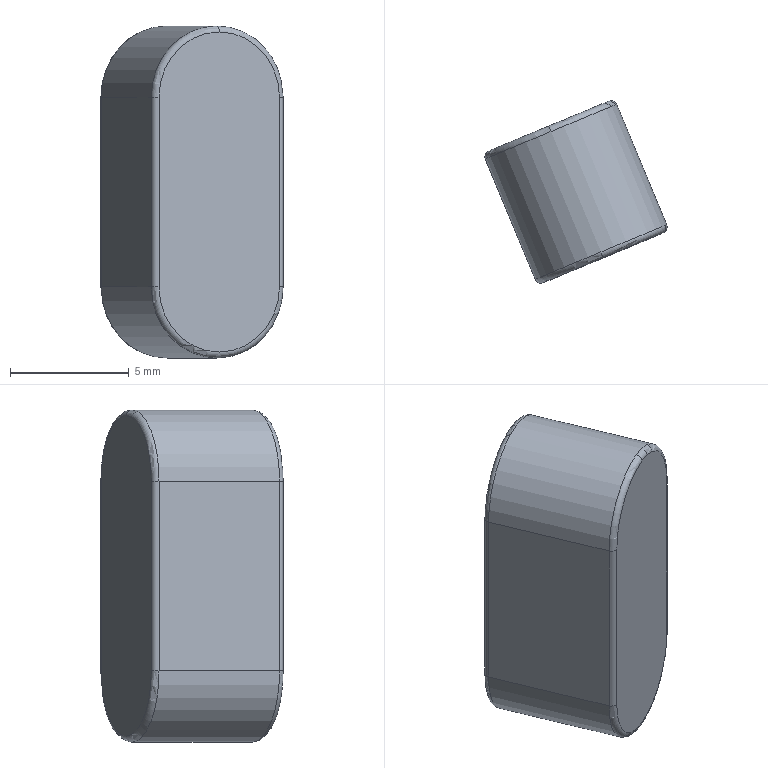Component | NX | GB_T_1096_2003_KEY_A_6X6X14 | 1 solid | 17 faces | box 7.69 x 7.69 x 14 mm | volume 457 mm3 | cylinder 7 | torus 6 | plane 4 | commonest cylinder face diameters 0.5 x4 6 x3
STEP:
#1=CARTESIAN_POINT('',(0.,0.,0.));
#2=DIRECTION('',(0.,0.,1.));
#3=DIRECTION('',(1.,0.,0.));
#4=AXIS2_PLACEMENT_3D('',#1,#2,#3);
#5=CARTESIAN_POINT('',(1.005,16.868,327.723));
#6=VERTEX_POINT('',#5);
#7=CARTESIAN_POINT('',(-1.536,15.814,324.973));
#8=VERTEX_POINT('',#7);
#9=CARTESIAN_POINT('',(1.005,16.868,324.973));
#10=DIRECTION('',(0.383,-0.9237,0.));
#11=DIRECTION('',(0.,0.,1.));
#12=AXIS2_PLACEMENT_3D('',#9,#10,#11);
#13=CIRCLE('',#12,2.75);
#14=CARTESIAN_POINT('',(0.9089,17.099,324.973));
#15=DIRECTION('',(-0.383,0.9237,0.));
#16=DIRECTION('',(0.,0.,-1.));
#17=AXIS2_PLACEMENT_3D('',#14,#15,#16);
#18=TOROIDAL_SURFACE('',#17,2.75,0.25);
#19=CARTESIAN_POINT('',(3.142,4.712));
#20=DIRECTION('',(-1.,-0.));
#21=VECTOR('',#20,1.);
#22=LINE('',#19,#21);
#23=(GEOMETRIC_REPRESENTATION_CONTEXT(2)PARAMETRIC_REPRESENTATION_CONTEXT()REPRESENTATION_CONTEXT('',''));
#24=DEFINITIONAL_REPRESENTATION('',(#22),#23);
#25=PCURVE('',#18,#24);
#26=CARTESIAN_POINT('',(1.005,16.868,316.973));
#27=DIRECTION('',(-0.383,0.9237,0.));
#28=DIRECTION('',(0.,0.,-1.));
#29=AXIS2_PLACEMENT_3D('',#26,#27,#28);
#30=PLANE('',#29);
#31=CARTESIAN_POINT('',(-10.75,0.));
#32=CARTESIAN_POINT('',(-10.75,4.763));
#33=CARTESIAN_POINT('',(-6.625,2.382));
#34=CARTESIAN_POINT('',(-2.5,0.));
#35=CARTESIAN_POINT('',(-6.625,-2.382));
#36=CARTESIAN_POINT('',(-10.75,-4.763));
#37=CARTESIAN_POINT('',(-10.75,0.));
#38=(BOUNDED_CURVE()B_SPLINE_CURVE(2,(#31,#32,#33,#34,#35,#36,#37),.UNSPECIFIED.,.T.,.F.)B_SPLINE_CURVE_WITH_KNOTS((1,2,2,2,2,1),(-2.094,0.,2.094,4.189,6.283,8.378),.UNSPECIFIED.)CURVE()GEOMETRIC_REPRESENTATION_ITEM()RATIONAL_B_SPLINE_CURVE((1.,0.5,1.,0.5,1.,0.5,1.))REPRESENTATION_ITEM(''));
#39=(GEOMETRIC_REPRESENTATION_CONTEXT(2)PARAMETRIC_REPRESENTATION_CONTEXT()REPRESENTATION_CONTEXT('',''));
#40=DEFINITIONAL_REPRESENTATION('',(#38),#39);
#41=PCURVE('',#30,#40);
#42=SURFACE_CURVE('',#13,(#25,#41),.PCURVE_S1.);
#43=EDGE_CURVE('',#6,#8,#42,.T.);
#44=ORIENTED_EDGE('',*,*,#43,.F.);
#45=CARTESIAN_POINT('',(0.9089,17.099,327.973));
#46=VERTEX_POINT('',#45);
#47=CARTESIAN_POINT('',(0.9089,17.099,327.723));
#48=DIRECTION('',(-0.9237,-0.383,0.));
#49=DIRECTION('',(0.383,-0.9237,0.));
#50=AXIS2_PLACEMENT_3D('',#47,#48,#49);
#51=CIRCLE('',#50,0.25);
#52=CARTESIAN_POINT('',(3.142,4.712));
#53=DIRECTION('',(0.,1.));
#54=VECTOR('',#53,1.);
#55=LINE('',#52,#54);
#56=(GEOMETRIC_REPRESENTATION_CONTEXT(2)PARAMETRIC_REPRESENTATION_CONTEXT()REPRESENTATION_CONTEXT('',''));
#57=DEFINITIONAL_REPRESENTATION('',(#55),#56);
#58=PCURVE('',#18,#57);
#59=CARTESIAN_POINT('',(0.9089,17.099,324.973));
#60=DIRECTION('',(-0.383,0.9237,0.));
#61=DIRECTION('',(0.,0.,-1.));
#62=AXIS2_PLACEMENT_3D('',#59,#60,#61);
#63=TOROIDAL_SURFACE('',#62,2.75,0.25);
#64=CARTESIAN_POINT('',(3.142,4.712));
#65=DIRECTION('',(0.,1.));
#66=VECTOR('',#65,1.);
#67=LINE('',#64,#66);
#68=(GEOMETRIC_REPRESENTATION_CONTEXT(2)PARAMETRIC_REPRESENTATION_CONTEXT()REPRESENTATION_CONTEXT('',''));
#69=DEFINITIONAL_REPRESENTATION('',(#67),#68);
#70=PCURVE('',#63,#69);
#71=SURFACE_CURVE('',#51,(#58,#70),.PCURVE_S1.);
#72=EDGE_CURVE('',#6,#46,#71,.T.);
#73=ORIENTED_EDGE('',*,*,#72,.T.);
#74=CARTESIAN_POINT('',(-1.862,15.949,324.973));
#75=VERTEX_POINT('',#74);
#76=CARTESIAN_POINT('',(0.9089,17.099,324.973));
#77=DIRECTION('',(-0.383,0.9237,0.));
#78=DIRECTION('',(0.,0.,1.));
#79=AXIS2_PLACEMENT_3D('',#76,#77,#78);
#80=CIRCLE('',#79,3.);
#81=CARTESIAN_POINT('',(-3.142,6.283));
#82=DIRECTION('',(1.,0.));
#83=VECTOR('',#82,1.);
#84=LINE('',#81,#83);
#85=(GEOMETRIC_REPRESENTATION_CONTEXT(2)PARAMETRIC_REPRESENTATION_CONTEXT()REPRESENTATION_CONTEXT('',''));
#86=DEFINITIONAL_REPRESENTATION('',(#84),#85);
#87=PCURVE('',#18,#86);
#88=CARTESIAN_POINT('',(-1.294,22.41,324.973));
#89=DIRECTION('',(0.383,-0.9237,0.));
#90=DIRECTION('',(0.,0.,1.));
#91=AXIS2_PLACEMENT_3D('',#88,#89,#90);
#92=CYLINDRICAL_SURFACE('',#91,3.);
#93=CARTESIAN_POINT('',(12.566,5.75));
#94=DIRECTION('',(-1.,-0.));
#95=VECTOR('',#94,1.);
#96=LINE('',#93,#95);
#97=(GEOMETRIC_REPRESENTATION_CONTEXT(2)PARAMETRIC_REPRESENTATION_CONTEXT()REPRESENTATION_CONTEXT('',''));
#98=DEFINITIONAL_REPRESENTATION('',(#96),#97);
#99=PCURVE('',#92,#98);
#100=SURFACE_CURVE('',#80,(#87,#99),.PCURVE_S1.);
#101=EDGE_CURVE('',#75,#46,#100,.T.);
#102=ORIENTED_EDGE('',*,*,#101,.F.);
#103=CARTESIAN_POINT('',(-1.631,16.045,324.973));
#104=DIRECTION('',(0.,0.,1.));
#105=DIRECTION('',(0.383,-0.9237,0.));
#106=AXIS2_PLACEMENT_3D('',#103,#104,#105);
#107=CIRCLE('',#106,0.25);
#108=CARTESIAN_POINT('',(1.571,10.996));
#109=DIRECTION('',(0.,-1.));
#110=VECTOR('',#109,1.);
#111=LINE('',#108,#110);
#112=(GEOMETRIC_REPRESENTATION_CONTEXT(2)PARAMETRIC_REPRESENTATION_CONTEXT()REPRESENTATION_CONTEXT('',''));
#113=DEFINITIONAL_REPRESENTATION('',(#111),#112);
#114=PCURVE('',#18,#113);
#115=CARTESIAN_POINT('',(-1.631,16.045,316.973));
#116=DIRECTION('',(0.,0.,1.));
#117=DIRECTION('',(-0.383,0.9237,0.));
#118=AXIS2_PLACEMENT_3D('',#115,#116,#117);
#119=CYLINDRICAL_SURFACE('',#118,0.25);
#120=CARTESIAN_POINT('',(-3.142,8.));
#121=DIRECTION('',(1.,0.));
#122=VECTOR('',#121,1.);
#123=LINE('',#120,#122);
#124=(GEOMETRIC_REPRESENTATION_CONTEXT(2)PARAMETRIC_REPRESENTATION_CONTEXT()REPRESENTATION_CONTEXT('',''));
#125=DEFINITIONAL_REPRESENTATION('',(#123),#124);
#126=PCURVE('',#119,#125);
#127=SURFACE_CURVE('',#107,(#114,#126),.PCURVE_S1.);
#128=EDGE_CURVE('',#75,#8,#127,.T.);
#129=ORIENTED_EDGE('',*,*,#128,.T.);
#130=EDGE_LOOP('',(#44,#73,#102,#129));
#131=FACE_BOUND('',#130,.T.);
#132=ADVANCED_FACE('',(#131),#18,.T.);
#133=CARTESIAN_POINT('',(-1.198,22.179,327.973));
#134=VERTEX_POINT('',#133);
#135=CARTESIAN_POINT('',(-3.969,21.03,324.973));
#136=VERTEX_POINT('',#135);
#137=CARTESIAN_POINT('',(-1.198,22.179,324.973));
#138=DIRECTION('',(0.383,-0.9237,0.));
#139=DIRECTION('',(0.,0.,1.));
#140=AXIS2_PLACEMENT_3D('',#137,#138,#139);
#141=CIRCLE('',#140,3.);
#142=CARTESIAN_POINT('',(-1.198,22.179,324.973));
#143=DIRECTION('',(-0.383,0.9237,0.));
#144=DIRECTION('',(0.,0.,-1.));
#145=AXIS2_PLACEMENT_3D('',#142,#143,#144);
#146=TOROIDAL_SURFACE('',#145,2.75,0.25);
#147=CARTESIAN_POINT('',(3.142,0.));
#148=DIRECTION('',(-1.,0.));
#149=VECTOR('',#148,1.);
#150=LINE('',#147,#149);
#151=(GEOMETRIC_REPRESENTATION_CONTEXT(2)PARAMETRIC_REPRESENTATION_CONTEXT()REPRESENTATION_CONTEXT('',''));
#152=DEFINITIONAL_REPRESENTATION('',(#150),#151);
#153=PCURVE('',#146,#152);
#154=CARTESIAN_POINT('',(6.283,0.25));
#155=DIRECTION('',(1.,-0.));
#156=VECTOR('',#155,1.);
#157=LINE('',#154,#156);
#158=(GEOMETRIC_REPRESENTATION_CONTEXT(2)PARAMETRIC_REPRESENTATION_CONTEXT()REPRESENTATION_CONTEXT('',''));
#159=DEFINITIONAL_REPRESENTATION('',(#157),#158);
#160=PCURVE('',#92,#159);
#161=SURFACE_CURVE('',#141,(#153,#160),.PCURVE_S1.);
#162=EDGE_CURVE('',#134,#136,#161,.T.);
#163=ORIENTED_EDGE('',*,*,#162,.F.);
#164=CARTESIAN_POINT('',(-1.294,22.41,327.723));
#165=VERTEX_POINT('',#164);
#166=CARTESIAN_POINT('',(-1.198,22.179,327.723));
#167=DIRECTION('',(-0.9237,-0.383,0.));
#168=DIRECTION('',(0.383,-0.9237,0.));
#169=AXIS2_PLACEMENT_3D('',#166,#167,#168);
#170=CIRCLE('',#169,0.25);
#171=CARTESIAN_POINT('',(3.142,-1.571));
#172=DIRECTION('',(0.,1.));
#173=VECTOR('',#172,1.);
#174=LINE('',#171,#173);
#175=(GEOMETRIC_REPRESENTATION_CONTEXT(2)PARAMETRIC_REPRESENTATION_CONTEXT()REPRESENTATION_CONTEXT('',''));
#176=DEFINITIONAL_REPRESENTATION('',(#174),#175);
#177=PCURVE('',#146,#176);
#178=CARTESIAN_POINT('',(-1.198,22.179,324.973));
#179=DIRECTION('',(-0.383,0.9237,0.));
#180=DIRECTION('',(0.,0.,-1.));
#181=AXIS2_PLACEMENT_3D('',#178,#179,#180);
#182=TOROIDAL_SURFACE('',#181,2.75,0.25);
#183=CARTESIAN_POINT('',(3.142,-1.571));
#184=DIRECTION('',(0.,1.));
#185=VECTOR('',#184,1.);
#186=LINE('',#183,#185);
#187=(GEOMETRIC_REPRESENTATION_CONTEXT(2)PARAMETRIC_REPRESENTATION_CONTEXT()REPRESENTATION_CONTEXT('',''));
#188=DEFINITIONAL_REPRESENTATION('',(#186),#187);
#189=PCURVE('',#182,#188);
#190=SURFACE_CURVE('',#170,(#177,#189),.PCURVE_S1.);
#191=EDGE_CURVE('',#134,#165,#190,.T.);
#192=ORIENTED_EDGE('',*,*,#191,.T.);
#193=CARTESIAN_POINT('',(-3.834,21.357,324.973));
#194=VERTEX_POINT('',#193);
#195=CARTESIAN_POINT('',(-1.294,22.41,324.973));
#196=DIRECTION('',(-0.383,0.9237,0.));
#197=DIRECTION('',(0.,0.,1.));
#198=AXIS2_PLACEMENT_3D('',#195,#196,#197);
#199=CIRCLE('',#198,2.75);
#200=CARTESIAN_POINT('',(-3.142,1.571));
#201=DIRECTION('',(1.,-0.));
#202=VECTOR('',#201,1.);
#203=LINE('',#200,#202);
#204=(GEOMETRIC_REPRESENTATION_CONTEXT(2)PARAMETRIC_REPRESENTATION_CONTEXT()REPRESENTATION_CONTEXT('',''));
#205=DEFINITIONAL_REPRESENTATION('',(#203),#204);
#206=PCURVE('',#146,#205);
#207=CARTESIAN_POINT('',(-1.294,22.41,316.973));
#208=DIRECTION('',(-0.383,0.9237,0.));
#209=DIRECTION('',(0.,0.,-1.));
#210=AXIS2_PLACEMENT_3D('',#207,#208,#209);
#211=PLANE('',#210);
#212=CARTESIAN_POINT('',(-8.,0.));
#213=DIRECTION('',(-1.,0.));
#214=AXIS2_PLACEMENT_2D('',#212,#213);
#215=CIRCLE('',#214,2.75);
#216=(GEOMETRIC_REPRESENTATION_CONTEXT(2)PARAMETRIC_REPRESENTATION_CONTEXT()REPRESENTATION_CONTEXT('',''));
#217=DEFINITIONAL_REPRESENTATION('',(#215),#216);
#218=PCURVE('',#211,#217);
#219=SURFACE_CURVE('',#199,(#206,#218),.PCURVE_S1.);
#220=EDGE_CURVE('',#194,#165,#219,.T.);
#221=ORIENTED_EDGE('',*,*,#220,.F.);
#222=CARTESIAN_POINT('',(-3.738,21.126,324.973));
#223=DIRECTION('',(0.,0.,1.));
#224=DIRECTION('',(0.383,-0.9237,0.));
#225=AXIS2_PLACEMENT_3D('',#222,#223,#224);
#226=CIRCLE('',#225,0.25);
#227=CARTESIAN_POINT('',(1.571,4.712));
#228=DIRECTION('',(0.,-1.));
#229=VECTOR('',#228,1.);
#230=LINE('',#227,#229);
#231=(GEOMETRIC_REPRESENTATION_CONTEXT(2)PARAMETRIC_REPRESENTATION_CONTEXT()REPRESENTATION_CONTEXT('',''));
#232=DEFINITIONAL_REPRESENTATION('',(#230),#231);
#233=PCURVE('',#146,#232);
#234=CARTESIAN_POINT('',(-3.738,21.126,316.973));
#235=DIRECTION('',(0.,0.,-1.));
#236=DIRECTION('',(0.383,-0.9237,0.));
#237=AXIS2_PLACEMENT_3D('',#234,#235,#236);
#238=CYLINDRICAL_SURFACE('',#237,0.25);
#239=CARTESIAN_POINT('',(6.283,-8.));
#240=DIRECTION('',(-1.,0.));
#241=VECTOR('',#240,1.);
#242=LINE('',#239,#241);
#243=(GEOMETRIC_REPRESENTATION_CONTEXT(2)PARAMETRIC_REPRESENTATION_CONTEXT()REPRESENTATION_CONTEXT('',''));
#244=DEFINITIONAL_REPRESENTATION('',(#242),#243);
#245=PCURVE('',#238,#244);
#246=SURFACE_CURVE('',#226,(#233,#245),.PCURVE_S1.);
#247=EDGE_CURVE('',#194,#136,#246,.T.);
#248=ORIENTED_EDGE('',*,*,#247,.T.);
#249=EDGE_LOOP('',(#163,#192,#221,#248));
#250=FACE_BOUND('',#249,.T.);
#251=ADVANCED_FACE('',(#250),#146,.T.);
#252=CARTESIAN_POINT('',(-3.969,21.03,316.973));
#253=VERTEX_POINT('',#252);
#254=CARTESIAN_POINT('',(-1.198,22.179,313.973));
#255=VERTEX_POINT('',#254);
#256=CARTESIAN_POINT('',(-1.198,22.179,316.973));
#257=DIRECTION('',(0.383,-0.9237,0.));
#258=DIRECTION('',(0.,0.,1.));
#259=AXIS2_PLACEMENT_3D('',#256,#257,#258);
#260=CIRCLE('',#259,3.);
#261=CARTESIAN_POINT('',(-1.294,22.41,316.973));
#262=DIRECTION('',(0.383,-0.9237,0.));
#263=DIRECTION('',(0.,0.,1.));
#264=AXIS2_PLACEMENT_3D('',#261,#262,#263);
#265=CYLINDRICAL_SURFACE('',#264,3.);
#266=CARTESIAN_POINT('',(-0.,0.25));
#267=DIRECTION('',(1.,0.));
#268=VECTOR('',#267,1.);
#269=LINE('',#266,#268);
#270=(GEOMETRIC_REPRESENTATION_CONTEXT(2)PARAMETRIC_REPRESENTATION_CONTEXT()REPRESENTATION_CONTEXT('',''));
#271=DEFINITIONAL_REPRESENTATION('',(#269),#270);
#272=PCURVE('',#265,#271);
#273=CARTESIAN_POINT('',(-1.198,22.179,316.973));
#274=DIRECTION('',(-0.383,0.9237,0.));
#275=DIRECTION('',(0.,0.,-1.));
#276=AXIS2_PLACEMENT_3D('',#273,#274,#275);
#277=TOROIDAL_SURFACE('',#276,2.75,0.25);
#278=CARTESIAN_POINT('',(9.425,0.));
#279=DIRECTION('',(-1.,0.));
#280=VECTOR('',#279,1.);
#281=LINE('',#278,#280);
#282=(GEOMETRIC_REPRESENTATION_CONTEXT(2)PARAMETRIC_REPRESENTATION_CONTEXT()REPRESENTATION_CONTEXT('',''));
#283=DEFINITIONAL_REPRESENTATION('',(#281),#282);
#284=PCURVE('',#277,#283);
#285=SURFACE_CURVE('',#260,(#272,#284),.PCURVE_S1.);
#286=EDGE_CURVE('',#253,#255,#285,.T.);
#287=ORIENTED_EDGE('',*,*,#286,.T.);
#288=CARTESIAN_POINT('',(0.9089,17.099,313.973));
#289=VERTEX_POINT('',#288);
#290=CARTESIAN_POINT('',(-1.294,22.41,313.973));
#291=DIRECTION('',(0.383,-0.9237,0.));
#292=VECTOR('',#291,1.);
#293=LINE('',#290,#292);
#294=CARTESIAN_POINT('',(3.142,0.));
#295=DIRECTION('',(0.,1.));
#296=VECTOR('',#295,1.);
#297=LINE('',#294,#296);
#298=(GEOMETRIC_REPRESENTATION_CONTEXT(2)PARAMETRIC_REPRESENTATION_CONTEXT()REPRESENTATION_CONTEXT('',''));
#299=DEFINITIONAL_REPRESENTATION('',(#297),#298);
#300=PCURVE('',#265,#299);
#301=CARTESIAN_POINT('',(-1.294,22.41,316.973));
#302=DIRECTION('',(0.383,-0.9237,0.));
#303=DIRECTION('',(0.,0.,1.));
#304=AXIS2_PLACEMENT_3D('',#301,#302,#303);
#305=CYLINDRICAL_SURFACE('',#304,3.);
#306=CARTESIAN_POINT('',(3.142,0.));
#307=DIRECTION('',(0.,1.));
#308=VECTOR('',#307,1.);
#309=LINE('',#306,#308);
#310=(GEOMETRIC_REPRESENTATION_CONTEXT(2)PARAMETRIC_REPRESENTATION_CONTEXT()REPRESENTATION_CONTEXT('',''));
#311=DEFINITIONAL_REPRESENTATION('',(#309),#310);
#312=PCURVE('',#305,#311);
#313=SURFACE_CURVE('',#293,(#300,#312),.PCURVE_S1.);
#314=EDGE_CURVE('',#255,#289,#313,.T.);
#315=ORIENTED_EDGE('',*,*,#314,.T.);
#316=CARTESIAN_POINT('',(-1.862,15.949,316.973));
#317=VERTEX_POINT('',#316);
#318=CARTESIAN_POINT('',(0.9089,17.099,316.973));
#319=DIRECTION('',(-0.383,0.9237,0.));
#320=DIRECTION('',(0.,0.,1.));
#321=AXIS2_PLACEMENT_3D('',#318,#319,#320);
#322=CIRCLE('',#321,3.);
#323=CARTESIAN_POINT('',(6.283,5.75));
#324=DIRECTION('',(-1.,0.));
#325=VECTOR('',#324,1.);
#326=LINE('',#323,#325);
#327=(GEOMETRIC_REPRESENTATION_CONTEXT(2)PARAMETRIC_REPRESENTATION_CONTEXT()REPRESENTATION_CONTEXT('',''));
#328=DEFINITIONAL_REPRESENTATION('',(#326),#327);
#329=PCURVE('',#265,#328);
#330=CARTESIAN_POINT('',(0.9089,17.099,316.973));
#331=DIRECTION('',(-0.383,0.9237,0.));
#332=DIRECTION('',(0.,0.,-1.));
#333=AXIS2_PLACEMENT_3D('',#330,#331,#332);
#334=TOROIDAL_SURFACE('',#333,2.75,0.25);
#335=CARTESIAN_POINT('',(3.142,6.283));
#336=DIRECTION('',(1.,0.));
#337=VECTOR('',#336,1.);
#338=LINE('',#335,#337);
#339=(GEOMETRIC_REPRESENTATION_CONTEXT(2)PARAMETRIC_REPRESENTATION_CONTEXT()REPRESENTATION_CONTEXT('',''));
#340=DEFINITIONAL_REPRESENTATION('',(#338),#339);
#341=PCURVE('',#334,#340);
#342=SURFACE_CURVE('',#322,(#329,#341),.PCURVE_S1.);
#343=EDGE_CURVE('',#289,#317,#342,.T.);
#344=ORIENTED_EDGE('',*,*,#343,.T.);
#345=CARTESIAN_POINT('',(-4.065,21.261,316.973));
#346=DIRECTION('',(0.383,-0.9237,0.));
#347=VECTOR('',#346,1.);
#348=LINE('',#345,#347);
#349=CARTESIAN_POINT('',(1.571,-0.));
#350=DIRECTION('',(0.,1.));
#351=VECTOR('',#350,1.);
#352=LINE('',#349,#351);
#353=(GEOMETRIC_REPRESENTATION_CONTEXT(2)PARAMETRIC_REPRESENTATION_CONTEXT()REPRESENTATION_CONTEXT('',''));
#354=DEFINITIONAL_REPRESENTATION('',(#352),#353);
#355=PCURVE('',#265,#354);
#356=CARTESIAN_POINT('',(-4.065,21.261,316.973));
#357=DIRECTION('',(0.9237,0.383,0.));
#358=DIRECTION('',(0.383,-0.9237,0.));
#359=AXIS2_PLACEMENT_3D('',#356,#357,#358);
#360=PLANE('',#359);
#361=CARTESIAN_POINT('',(0.,0.));
#362=DIRECTION('',(1.,0.));
#363=VECTOR('',#362,1.);
#364=LINE('',#361,#363);
#365=(GEOMETRIC_REPRESENTATION_CONTEXT(2)PARAMETRIC_REPRESENTATION_CONTEXT()REPRESENTATION_CONTEXT('',''));
#366=DEFINITIONAL_REPRESENTATION('',(#364),#365);
#367=PCURVE('',#360,#366);
#368=SURFACE_CURVE('',#348,(#355,#367),.PCURVE_S1.);
#369=EDGE_CURVE('',#253,#317,#368,.T.);
#370=ORIENTED_EDGE('',*,*,#369,.F.);
#371=EDGE_LOOP('',(#287,#315,#344,#370));
#372=FACE_BOUND('',#371,.T.);
#373=ADVANCED_FACE('',(#372),#265,.T.);
#374=ORIENTED_EDGE('',*,*,#314,.F.);
#375=CARTESIAN_POINT('',(1.573,23.328,316.973));
#376=VERTEX_POINT('',#375);
#377=CARTESIAN_POINT('',(-1.198,22.179,316.973));
#378=DIRECTION('',(0.383,-0.9237,0.));
#379=DIRECTION('',(0.,0.,1.));
#380=AXIS2_PLACEMENT_3D('',#377,#378,#379);
#381=CIRCLE('',#380,3.);
#382=CARTESIAN_POINT('',(-0.,0.25));
#383=DIRECTION('',(1.,0.));
#384=VECTOR('',#383,1.);
#385=LINE('',#382,#384);
#386=(GEOMETRIC_REPRESENTATION_CONTEXT(2)PARAMETRIC_REPRESENTATION_CONTEXT()REPRESENTATION_CONTEXT('',''));
#387=DEFINITIONAL_REPRESENTATION('',(#385),#386);
#388=PCURVE('',#305,#387);
#389=CARTESIAN_POINT('',(9.425,0.));
#390=DIRECTION('',(-1.,0.));
#391=VECTOR('',#390,1.);
#392=LINE('',#389,#391);
#393=(GEOMETRIC_REPRESENTATION_CONTEXT(2)PARAMETRIC_REPRESENTATION_CONTEXT()REPRESENTATION_CONTEXT('',''));
#394=DEFINITIONAL_REPRESENTATION('',(#392),#393);
#395=PCURVE('',#277,#394);
#396=SURFACE_CURVE('',#381,(#388,#395),.PCURVE_S1.);
#397=EDGE_CURVE('',#255,#376,#396,.T.);
#398=ORIENTED_EDGE('',*,*,#397,.T.);
#399=CARTESIAN_POINT('',(3.68,18.248,316.973));
#400=VERTEX_POINT('',#399);
#401=CARTESIAN_POINT('',(1.478,23.559,316.973));
#402=DIRECTION('',(0.383,-0.9237,0.));
#403=VECTOR('',#402,1.);
#404=LINE('',#401,#403);
#405=CARTESIAN_POINT('',(4.712,0.));
#406=DIRECTION('',(0.,1.));
#407=VECTOR('',#406,1.);
#408=LINE('',#405,#407);
#409=(GEOMETRIC_REPRESENTATION_CONTEXT(2)PARAMETRIC_REPRESENTATION_CONTEXT()REPRESENTATION_CONTEXT('',''));
#410=DEFINITIONAL_REPRESENTATION('',(#408),#409);
#411=PCURVE('',#305,#410);
#412=CARTESIAN_POINT('',(1.478,23.559,316.973));
#413=DIRECTION('',(-0.9237,-0.383,0.));
#414=DIRECTION('',(-0.383,0.9237,0.));
#415=AXIS2_PLACEMENT_3D('',#412,#413,#414);
#416=PLANE('',#415);
#417=CARTESIAN_POINT('',(0.,0.));
#418=DIRECTION('',(-1.,0.));
#419=VECTOR('',#418,1.);
#420=LINE('',#417,#419);
#421=(GEOMETRIC_REPRESENTATION_CONTEXT(2)PARAMETRIC_REPRESENTATION_CONTEXT()REPRESENTATION_CONTEXT('',''));
#422=DEFINITIONAL_REPRESENTATION('',(#420),#421);
#423=PCURVE('',#416,#422);
#424=SURFACE_CURVE('',#404,(#411,#423),.PCURVE_S1.);
#425=EDGE_CURVE('',#376,#400,#424,.T.);
#426=ORIENTED_EDGE('',*,*,#425,.T.);
#427=CARTESIAN_POINT('',(0.9089,17.099,316.973));
#428=DIRECTION('',(-0.383,0.9237,0.));
#429=DIRECTION('',(0.,0.,1.));
#430=AXIS2_PLACEMENT_3D('',#427,#428,#429);
#431=CIRCLE('',#430,3.);
#432=CARTESIAN_POINT('',(6.283,5.75));
#433=DIRECTION('',(-1.,0.));
#434=VECTOR('',#433,1.);
#435=LINE('',#432,#434);
#436=(GEOMETRIC_REPRESENTATION_CONTEXT(2)PARAMETRIC_REPRESENTATION_CONTEXT()REPRESENTATION_CONTEXT('',''));
#437=DEFINITIONAL_REPRESENTATION('',(#435),#436);
#438=PCURVE('',#305,#437);
#439=CARTESIAN_POINT('',(3.142,6.283));
#440=DIRECTION('',(1.,0.));
#441=VECTOR('',#440,1.);
#442=LINE('',#439,#441);
#443=(GEOMETRIC_REPRESENTATION_CONTEXT(2)PARAMETRIC_REPRESENTATION_CONTEXT()REPRESENTATION_CONTEXT('',''));
#444=DEFINITIONAL_REPRESENTATION('',(#442),#443);
#445=PCURVE('',#334,#444);
#446=SURFACE_CURVE('',#431,(#438,#445),.PCURVE_S1.);
#447=EDGE_CURVE('',#400,#289,#446,.T.);
#448=ORIENTED_EDGE('',*,*,#447,.T.);
#449=EDGE_LOOP('',(#374,#398,#426,#448));
#450=FACE_BOUND('',#449,.T.);
#451=ADVANCED_FACE('',(#450),#305,.T.);
#452=CARTESIAN_POINT('',(-4.065,21.261,324.973));
#453=DIRECTION('',(0.383,-0.9237,0.));
#454=VECTOR('',#453,1.);
#455=LINE('',#452,#454);
#456=CARTESIAN_POINT('',(-0.,-8.));
#457=DIRECTION('',(1.,0.));
#458=VECTOR('',#457,1.);
#459=LINE('',#456,#458);
#460=(GEOMETRIC_REPRESENTATION_CONTEXT(2)PARAMETRIC_REPRESENTATION_CONTEXT()REPRESENTATION_CONTEXT('',''));
#461=DEFINITIONAL_REPRESENTATION('',(#459),#460);
#462=PCURVE('',#360,#461);
#463=CARTESIAN_POINT('',(7.854,-0.));
#464=DIRECTION('',(0.,1.));
#465=VECTOR('',#464,1.);
#466=LINE('',#463,#465);
#467=(GEOMETRIC_REPRESENTATION_CONTEXT(2)PARAMETRIC_REPRESENTATION_CONTEXT()REPRESENTATION_CONTEXT('',''));
#468=DEFINITIONAL_REPRESENTATION('',(#466),#467);
#469=PCURVE('',#92,#468);
#470=SURFACE_CURVE('',#455,(#462,#469),.PCURVE_S1.);
#471=EDGE_CURVE('',#136,#75,#470,.T.);
#472=ORIENTED_EDGE('',*,*,#471,.F.);
#473=CARTESIAN_POINT('',(-3.969,21.03,316.973));
#474=DIRECTION('',(0.,0.,-1.));
#475=VECTOR('',#474,1.);
#476=LINE('',#473,#475);
#477=CARTESIAN_POINT('',(0.25,0.));
#478=DIRECTION('',(0.,1.));
#479=VECTOR('',#478,1.);
#480=LINE('',#477,#479);
#481=(GEOMETRIC_REPRESENTATION_CONTEXT(2)PARAMETRIC_REPRESENTATION_CONTEXT()REPRESENTATION_CONTEXT('',''));
#482=DEFINITIONAL_REPRESENTATION('',(#480),#481);
#483=PCURVE('',#360,#482);
#484=CARTESIAN_POINT('',(1.571,0.));
#485=DIRECTION('',(0.,1.));
#486=VECTOR('',#485,1.);
#487=LINE('',#484,#486);
#488=(GEOMETRIC_REPRESENTATION_CONTEXT(2)PARAMETRIC_REPRESENTATION_CONTEXT()REPRESENTATION_CONTEXT('',''));
#489=DEFINITIONAL_REPRESENTATION('',(#487),#488);
#490=PCURVE('',#238,#489);
#491=SURFACE_CURVE('',#476,(#483,#490),.PCURVE_S1.);
#492=EDGE_CURVE('',#136,#253,#491,.T.);
#493=ORIENTED_EDGE('',*,*,#492,.T.);
#494=ORIENTED_EDGE('',*,*,#369,.T.);
#495=CARTESIAN_POINT('',(-1.862,15.949,316.973));
#496=DIRECTION('',(0.,0.,1.));
#497=VECTOR('',#496,1.);
#498=LINE('',#495,#497);
#499=CARTESIAN_POINT('',(5.75,0.));
#500=DIRECTION('',(0.,-1.));
#501=VECTOR('',#500,1.);
#502=LINE('',#499,#501);
#503=(GEOMETRIC_REPRESENTATION_CONTEXT(2)PARAMETRIC_REPRESENTATION_CONTEXT()REPRESENTATION_CONTEXT('',''));
#504=DEFINITIONAL_REPRESENTATION('',(#502),#503);
#505=PCURVE('',#360,#504);
#506=CARTESIAN_POINT('',(1.571,0.));
#507=DIRECTION('',(0.,1.));
#508=VECTOR('',#507,1.);
#509=LINE('',#506,#508);
#510=(GEOMETRIC_REPRESENTATION_CONTEXT(2)PARAMETRIC_REPRESENTATION_CONTEXT()REPRESENTATION_CONTEXT('',''));
#511=DEFINITIONAL_REPRESENTATION('',(#509),#510);
#512=PCURVE('',#119,#511);
#513=SURFACE_CURVE('',#498,(#505,#512),.PCURVE_S1.);
#514=EDGE_CURVE('',#317,#75,#513,.T.);
#515=ORIENTED_EDGE('',*,*,#514,.T.);
#516=EDGE_LOOP('',(#472,#493,#494,#515));
#517=FACE_BOUND('',#516,.T.);
#518=ADVANCED_FACE('',(#517),#360,.F.);
#519=CARTESIAN_POINT('',(1.573,23.328,324.973));
#520=VERTEX_POINT('',#519);
#521=CARTESIAN_POINT('',(3.68,18.248,324.973));
#522=VERTEX_POINT('',#521);
#523=CARTESIAN_POINT('',(1.478,23.559,324.973));
#524=DIRECTION('',(0.383,-0.9237,0.));
#525=VECTOR('',#524,1.);
#526=LINE('',#523,#525);
#527=CARTESIAN_POINT('',(4.712,0.));
#528=DIRECTION('',(0.,1.));
#529=VECTOR('',#528,1.);
#530=LINE('',#527,#529);
#531=(GEOMETRIC_REPRESENTATION_CONTEXT(2)PARAMETRIC_REPRESENTATION_CONTEXT()REPRESENTATION_CONTEXT('',''));
#532=DEFINITIONAL_REPRESENTATION('',(#530),#531);
#533=PCURVE('',#92,#532);
#534=CARTESIAN_POINT('',(0.,-8.));
#535=DIRECTION('',(-1.,0.));
#536=VECTOR('',#535,1.);
#537=LINE('',#534,#536);
#538=(GEOMETRIC_REPRESENTATION_CONTEXT(2)PARAMETRIC_REPRESENTATION_CONTEXT()REPRESENTATION_CONTEXT('',''));
#539=DEFINITIONAL_REPRESENTATION('',(#537),#538);
#540=PCURVE('',#416,#539);
#541=SURFACE_CURVE('',#526,(#533,#540),.PCURVE_S1.);
#542=EDGE_CURVE('',#520,#522,#541,.T.);
#543=ORIENTED_EDGE('',*,*,#542,.F.);
#544=CARTESIAN_POINT('',(-1.198,22.179,324.973));
#545=DIRECTION('',(0.383,-0.9237,0.));
#546=DIRECTION('',(0.,0.,1.));
#547=AXIS2_PLACEMENT_3D('',#544,#545,#546);
#548=CIRCLE('',#547,3.);
#549=CARTESIAN_POINT('',(0.,0.25));
#550=DIRECTION('',(1.,-0.));
#551=VECTOR('',#550,1.);
#552=LINE('',#549,#551);
#553=(GEOMETRIC_REPRESENTATION_CONTEXT(2)PARAMETRIC_REPRESENTATION_CONTEXT()REPRESENTATION_CONTEXT('',''));
#554=DEFINITIONAL_REPRESENTATION('',(#552),#553);
#555=PCURVE('',#92,#554);
#556=CARTESIAN_POINT('',(9.425,0.));
#557=DIRECTION('',(-1.,0.));
#558=VECTOR('',#557,1.);
#559=LINE('',#556,#558);
#560=(GEOMETRIC_REPRESENTATION_CONTEXT(2)PARAMETRIC_REPRESENTATION_CONTEXT()REPRESENTATION_CONTEXT('',''));
#561=DEFINITIONAL_REPRESENTATION('',(#559),#560);
#562=PCURVE('',#182,#561);
#563=SURFACE_CURVE('',#548,(#555,#562),.PCURVE_S1.);
#564=EDGE_CURVE('',#520,#134,#563,.T.);
#565=ORIENTED_EDGE('',*,*,#564,.T.);
#566=ORIENTED_EDGE('',*,*,#162,.T.);
#567=ORIENTED_EDGE('',*,*,#471,.T.);
#568=ORIENTED_EDGE('',*,*,#101,.T.);
#569=CARTESIAN_POINT('',(0.9089,17.099,324.973));
#570=DIRECTION('',(-0.383,0.9237,0.));
#571=DIRECTION('',(0.,0.,1.));
#572=AXIS2_PLACEMENT_3D('',#569,#570,#571);
#573=CIRCLE('',#572,3.);
#574=CARTESIAN_POINT('',(6.283,5.75));
#575=DIRECTION('',(-1.,0.));
#576=VECTOR('',#575,1.);
#577=LINE('',#574,#576);
#578=(GEOMETRIC_REPRESENTATION_CONTEXT(2)PARAMETRIC_REPRESENTATION_CONTEXT()REPRESENTATION_CONTEXT('',''));
#579=DEFINITIONAL_REPRESENTATION('',(#577),#578);
#580=PCURVE('',#92,#579);
#581=CARTESIAN_POINT('',(3.142,6.283));
#582=DIRECTION('',(1.,0.));
#583=VECTOR('',#582,1.);
#584=LINE('',#581,#583);
#585=(GEOMETRIC_REPRESENTATION_CONTEXT(2)PARAMETRIC_REPRESENTATION_CONTEXT()REPRESENTATION_CONTEXT('',''));
#586=DEFINITIONAL_REPRESENTATION('',(#584),#585);
#587=PCURVE('',#63,#586);
#588=SURFACE_CURVE('',#573,(#580,#587),.PCURVE_S1.);
#589=EDGE_CURVE('',#46,#522,#588,.T.);
#590=ORIENTED_EDGE('',*,*,#589,.T.);
#591=EDGE_LOOP('',(#543,#565,#566,#567,#568,#590));
#592=FACE_BOUND('',#591,.T.);
#593=ADVANCED_FACE('',(#592),#92,.T.);
#594=ORIENTED_EDGE('',*,*,#425,.F.);
#595=CARTESIAN_POINT('',(1.573,23.328,324.973));
#596=DIRECTION('',(0.,0.,1.));
#597=VECTOR('',#596,1.);
#598=LINE('',#595,#597);
#599=CARTESIAN_POINT('',(-0.25,-8.));
#600=DIRECTION('',(0.,-1.));
#601=VECTOR('',#600,1.);
#602=LINE('',#599,#601);
#603=(GEOMETRIC_REPRESENTATION_CONTEXT(2)PARAMETRIC_REPRESENTATION_CONTEXT()REPRESENTATION_CONTEXT('',''));
#604=DEFINITIONAL_REPRESENTATION('',(#602),#603);
#605=PCURVE('',#416,#604);
#606=CARTESIAN_POINT('',(1.342,23.232,316.973));
#607=DIRECTION('',(0.,0.,1.));
#608=DIRECTION('',(-0.383,0.9237,0.));
#609=AXIS2_PLACEMENT_3D('',#606,#607,#608);
#610=CYLINDRICAL_SURFACE('',#609,0.25);
#611=CARTESIAN_POINT('',(4.712,8.));
#612=DIRECTION('',(0.,1.));
#613=VECTOR('',#612,1.);
#614=LINE('',#611,#613);
#615=(GEOMETRIC_REPRESENTATION_CONTEXT(2)PARAMETRIC_REPRESENTATION_CONTEXT()REPRESENTATION_CONTEXT('',''));
#616=DEFINITIONAL_REPRESENTATION('',(#614),#615);
#617=PCURVE('',#610,#616);
#618=SURFACE_CURVE('',#598,(#605,#617),.PCURVE_S1.);
#619=EDGE_CURVE('',#376,#520,#618,.T.);
#620=ORIENTED_EDGE('',*,*,#619,.T.);
#621=ORIENTED_EDGE('',*,*,#542,.T.);
#622=CARTESIAN_POINT('',(3.68,18.248,316.973));
#623=DIRECTION('',(0.,0.,-1.));
#624=VECTOR('',#623,1.);
#625=LINE('',#622,#624);
#626=CARTESIAN_POINT('',(-5.75,0.));
#627=DIRECTION('',(0.,1.));
#628=VECTOR('',#627,1.);
#629=LINE('',#626,#628);
#630=(GEOMETRIC_REPRESENTATION_CONTEXT(2)PARAMETRIC_REPRESENTATION_CONTEXT()REPRESENTATION_CONTEXT('',''));
#631=DEFINITIONAL_REPRESENTATION('',(#629),#630);
#632=PCURVE('',#416,#631);
#633=CARTESIAN_POINT('',(3.449,18.152,316.973));
#634=DIRECTION('',(0.,0.,-1.));
#635=DIRECTION('',(0.383,-0.9237,0.));
#636=AXIS2_PLACEMENT_3D('',#633,#634,#635);
#637=CYLINDRICAL_SURFACE('',#636,0.25);
#638=CARTESIAN_POINT('',(4.712,0.));
#639=DIRECTION('',(0.,1.));
#640=VECTOR('',#639,1.);
#641=LINE('',#638,#640);
#642=(GEOMETRIC_REPRESENTATION_CONTEXT(2)PARAMETRIC_REPRESENTATION_CONTEXT()REPRESENTATION_CONTEXT('',''));
#643=DEFINITIONAL_REPRESENTATION('',(#641),#642);
#644=PCURVE('',#637,#643);
#645=SURFACE_CURVE('',#625,(#632,#644),.PCURVE_S1.);
#646=EDGE_CURVE('',#522,#400,#645,.T.);
#647=ORIENTED_EDGE('',*,*,#646,.T.);
#648=EDGE_LOOP('',(#594,#620,#621,#647));
#649=FACE_BOUND('',#648,.T.);
#650=ADVANCED_FACE('',(#649),#416,.F.);
#651=CARTESIAN_POINT('',(-3.834,21.357,316.973));
#652=VERTEX_POINT('',#651);
#653=CARTESIAN_POINT('',(-3.834,21.357,324.973));
#654=DIRECTION('',(0.,0.,1.));
#655=VECTOR('',#654,1.);
#656=LINE('',#653,#655);
#657=CARTESIAN_POINT('',(-8.,2.75));
#658=DIRECTION('',(-1.,0.));
#659=VECTOR('',#658,1.);
#660=LINE('',#657,#659);
#661=(GEOMETRIC_REPRESENTATION_CONTEXT(2)PARAMETRIC_REPRESENTATION_CONTEXT()REPRESENTATION_CONTEXT('',''));
#662=DEFINITIONAL_REPRESENTATION('',(#660),#661);
#663=PCURVE('',#211,#662);
#664=CARTESIAN_POINT('',(3.142,-8.));
#665=DIRECTION('',(0.,-1.));
#666=VECTOR('',#665,1.);
#667=LINE('',#664,#666);
#668=(GEOMETRIC_REPRESENTATION_CONTEXT(2)PARAMETRIC_REPRESENTATION_CONTEXT()REPRESENTATION_CONTEXT('',''));
#669=DEFINITIONAL_REPRESENTATION('',(#667),#668);
#670=PCURVE('',#238,#669);
#671=SURFACE_CURVE('',#656,(#663,#670),.PCURVE_S1.);
#672=EDGE_CURVE('',#652,#194,#671,.T.);
#673=ORIENTED_EDGE('',*,*,#672,.T.);
#674=ORIENTED_EDGE('',*,*,#220,.T.);
#675=CARTESIAN_POINT('',(1.247,23.463,324.973));
#676=VERTEX_POINT('',#675);
#677=CARTESIAN_POINT('',(-1.294,22.41,324.973));
#678=DIRECTION('',(-0.383,0.9237,0.));
#679=DIRECTION('',(0.,0.,1.));
#680=AXIS2_PLACEMENT_3D('',#677,#678,#679);
#681=CIRCLE('',#680,2.75);
#682=CARTESIAN_POINT('',(-8.,0.));
#683=DIRECTION('',(-1.,0.));
#684=AXIS2_PLACEMENT_2D('',#682,#683);
#685=CIRCLE('',#684,2.75);
#686=(GEOMETRIC_REPRESENTATION_CONTEXT(2)PARAMETRIC_REPRESENTATION_CONTEXT()REPRESENTATION_CONTEXT('',''));
#687=DEFINITIONAL_REPRESENTATION('',(#685),#686);
#688=PCURVE('',#211,#687);
#689=CARTESIAN_POINT('',(3.142,1.571));
#690=DIRECTION('',(1.,-0.));
#691=VECTOR('',#690,1.);
#692=LINE('',#689,#691);
#693=(GEOMETRIC_REPRESENTATION_CONTEXT(2)PARAMETRIC_REPRESENTATION_CONTEXT()REPRESENTATION_CONTEXT('',''));
#694=DEFINITIONAL_REPRESENTATION('',(#692),#693);
#695=PCURVE('',#182,#694);
#696=SURFACE_CURVE('',#681,(#688,#695),.PCURVE_S1.);
#697=EDGE_CURVE('',#165,#676,#696,.T.);
#698=ORIENTED_EDGE('',*,*,#697,.T.);
#699=CARTESIAN_POINT('',(1.247,23.463,316.973));
#700=VERTEX_POINT('',#699);
#701=CARTESIAN_POINT('',(1.247,23.463,316.973));
#702=DIRECTION('',(0.,0.,-1.));
#703=VECTOR('',#702,1.);
#704=LINE('',#701,#703);
#705=CARTESIAN_POINT('',(0.,-2.75));
#706=DIRECTION('',(1.,0.));
#707=VECTOR('',#706,1.);
#708=LINE('',#705,#707);
#709=(GEOMETRIC_REPRESENTATION_CONTEXT(2)PARAMETRIC_REPRESENTATION_CONTEXT()REPRESENTATION_CONTEXT('',''));
#710=DEFINITIONAL_REPRESENTATION('',(#708),#709);
#711=PCURVE('',#211,#710);
#712=CARTESIAN_POINT('',(6.283,0.));
#713=DIRECTION('',(0.,-1.));
#714=VECTOR('',#713,1.);
#715=LINE('',#712,#714);
#716=(GEOMETRIC_REPRESENTATION_CONTEXT(2)PARAMETRIC_REPRESENTATION_CONTEXT()REPRESENTATION_CONTEXT('',''));
#717=DEFINITIONAL_REPRESENTATION('',(#715),#716);
#718=PCURVE('',#610,#717);
#719=SURFACE_CURVE('',#704,(#711,#718),.PCURVE_S1.);
#720=EDGE_CURVE('',#676,#700,#719,.T.);
#721=ORIENTED_EDGE('',*,*,#720,.T.);
#722=CARTESIAN_POINT('',(-1.294,22.41,316.973));
#723=DIRECTION('',(-0.383,0.9237,0.));
#724=DIRECTION('',(0.,0.,1.));
#725=AXIS2_PLACEMENT_3D('',#722,#723,#724);
#726=CIRCLE('',#725,2.75);
#727=CARTESIAN_POINT('',(0.,0.));
#728=DIRECTION('',(-1.,0.));
#729=AXIS2_PLACEMENT_2D('',#727,#728);
#730=CIRCLE('',#729,2.75);
#731=(GEOMETRIC_REPRESENTATION_CONTEXT(2)PARAMETRIC_REPRESENTATION_CONTEXT()REPRESENTATION_CONTEXT('',''));
#732=DEFINITIONAL_REPRESENTATION('',(#730),#731);
#733=PCURVE('',#211,#732);
#734=CARTESIAN_POINT('',(3.142,1.571));
#735=DIRECTION('',(1.,0.));
#736=VECTOR('',#735,1.);
#737=LINE('',#734,#736);
#738=(GEOMETRIC_REPRESENTATION_CONTEXT(2)PARAMETRIC_REPRESENTATION_CONTEXT()REPRESENTATION_CONTEXT('',''));
#739=DEFINITIONAL_REPRESENTATION('',(#737),#738);
#740=PCURVE('',#277,#739);
#741=SURFACE_CURVE('',#726,(#733,#740),.PCURVE_S1.);
#742=EDGE_CURVE('',#700,#652,#741,.T.);
#743=ORIENTED_EDGE('',*,*,#742,.T.);
#744=EDGE_LOOP('',(#673,#674,#698,#721,#743));
#745=FACE_BOUND('',#744,.T.);
#746=ADVANCED_FACE('',(#745),#211,.T.);
#747=CARTESIAN_POINT('',(3.545,17.921,316.973));
#748=VERTEX_POINT('',#747);
#749=CARTESIAN_POINT('',(3.545,17.921,324.973));
#750=VERTEX_POINT('',#749);
#751=CARTESIAN_POINT('',(3.545,17.921,316.973));
#752=DIRECTION('',(0.,0.,1.));
#753=VECTOR('',#752,1.);
#754=LINE('',#751,#753);
#755=CARTESIAN_POINT('',(0.,-2.75));
#756=DIRECTION('',(-1.,0.));
#757=VECTOR('',#756,1.);
#758=LINE('',#755,#757);
#759=(GEOMETRIC_REPRESENTATION_CONTEXT(2)PARAMETRIC_REPRESENTATION_CONTEXT()REPRESENTATION_CONTEXT('',''));
#760=DEFINITIONAL_REPRESENTATION('',(#758),#759);
#761=PCURVE('',#30,#760);
#762=CARTESIAN_POINT('',(6.283,0.));
#763=DIRECTION('',(0.,-1.));
#764=VECTOR('',#763,1.);
#765=LINE('',#762,#764);
#766=(GEOMETRIC_REPRESENTATION_CONTEXT(2)PARAMETRIC_REPRESENTATION_CONTEXT()REPRESENTATION_CONTEXT('',''));
#767=DEFINITIONAL_REPRESENTATION('',(#765),#766);
#768=PCURVE('',#637,#767);
#769=SURFACE_CURVE('',#754,(#761,#768),.PCURVE_S1.);
#770=EDGE_CURVE('',#748,#750,#769,.T.);
#771=ORIENTED_EDGE('',*,*,#770,.T.);
#772=CARTESIAN_POINT('',(1.005,16.868,324.973));
#773=DIRECTION('',(0.383,-0.9237,0.));
#774=DIRECTION('',(0.,0.,1.));
#775=AXIS2_PLACEMENT_3D('',#772,#773,#774);
#776=CIRCLE('',#775,2.75);
#777=CARTESIAN_POINT('',(-10.75,0.));
#778=CARTESIAN_POINT('',(-10.75,4.763));
#779=CARTESIAN_POINT('',(-6.625,2.382));
#780=CARTESIAN_POINT('',(-2.5,0.));
#781=CARTESIAN_POINT('',(-6.625,-2.382));
#782=CARTESIAN_POINT('',(-10.75,-4.763));
#783=CARTESIAN_POINT('',(-10.75,0.));
#784=(BOUNDED_CURVE()B_SPLINE_CURVE(2,(#777,#778,#779,#780,#781,#782,#783),.UNSPECIFIED.,.T.,.F.)B_SPLINE_CURVE_WITH_KNOTS((1,2,2,2,2,1),(-2.094,0.,2.094,4.189,6.283,8.378),.UNSPECIFIED.)CURVE()GEOMETRIC_REPRESENTATION_ITEM()RATIONAL_B_SPLINE_CURVE((1.,0.5,1.,0.5,1.,0.5,1.))REPRESENTATION_ITEM(''));
#785=(GEOMETRIC_REPRESENTATION_CONTEXT(2)PARAMETRIC_REPRESENTATION_CONTEXT()REPRESENTATION_CONTEXT('',''));
#786=DEFINITIONAL_REPRESENTATION('',(#784),#785);
#787=PCURVE('',#30,#786);
#788=CARTESIAN_POINT('',(9.425,4.712));
#789=DIRECTION('',(-1.,-0.));
#790=VECTOR('',#789,1.);
#791=LINE('',#788,#790);
#792=(GEOMETRIC_REPRESENTATION_CONTEXT(2)PARAMETRIC_REPRESENTATION_CONTEXT()REPRESENTATION_CONTEXT('',''));
#793=DEFINITIONAL_REPRESENTATION('',(#791),#792);
#794=PCURVE('',#63,#793);
#795=SURFACE_CURVE('',#776,(#787,#794),.PCURVE_S1.);
#796=EDGE_CURVE('',#750,#6,#795,.T.);
#797=ORIENTED_EDGE('',*,*,#796,.T.);
#798=ORIENTED_EDGE('',*,*,#43,.T.);
#799=CARTESIAN_POINT('',(-1.536,15.814,316.973));
#800=VERTEX_POINT('',#799);
#801=CARTESIAN_POINT('',(-1.536,15.814,316.973));
#802=DIRECTION('',(0.,0.,-1.));
#803=VECTOR('',#802,1.);
#804=LINE('',#801,#803);
#805=CARTESIAN_POINT('',(0.,2.75));
#806=DIRECTION('',(1.,0.));
#807=VECTOR('',#806,1.);
#808=LINE('',#805,#807);
#809=(GEOMETRIC_REPRESENTATION_CONTEXT(2)PARAMETRIC_REPRESENTATION_CONTEXT()REPRESENTATION_CONTEXT('',''));
#810=DEFINITIONAL_REPRESENTATION('',(#808),#809);
#811=PCURVE('',#30,#810);
#812=CARTESIAN_POINT('',(3.142,0.));
#813=DIRECTION('',(0.,-1.));
#814=VECTOR('',#813,1.);
#815=LINE('',#812,#814);
#816=(GEOMETRIC_REPRESENTATION_CONTEXT(2)PARAMETRIC_REPRESENTATION_CONTEXT()REPRESENTATION_CONTEXT('',''));
#817=DEFINITIONAL_REPRESENTATION('',(#815),#816);
#818=PCURVE('',#119,#817);
#819=SURFACE_CURVE('',#804,(#811,#818),.PCURVE_S1.);
#820=EDGE_CURVE('',#8,#800,#819,.T.);
#821=ORIENTED_EDGE('',*,*,#820,.T.);
#822=CARTESIAN_POINT('',(1.005,16.868,316.973));
#823=DIRECTION('',(0.383,-0.9237,0.));
#824=DIRECTION('',(0.,0.,1.));
#825=AXIS2_PLACEMENT_3D('',#822,#823,#824);
#826=CIRCLE('',#825,2.75);
#827=CARTESIAN_POINT('',(-2.75,-0.));
#828=CARTESIAN_POINT('',(-2.75,4.763));
#829=CARTESIAN_POINT('',(1.375,2.382));
#830=CARTESIAN_POINT('',(5.5,0.));
#831=CARTESIAN_POINT('',(1.375,-2.382));
#832=CARTESIAN_POINT('',(-2.75,-4.763));
#833=CARTESIAN_POINT('',(-2.75,-0.));
#834=(BOUNDED_CURVE()B_SPLINE_CURVE(2,(#827,#828,#829,#830,#831,#832,#833),.UNSPECIFIED.,.T.,.F.)B_SPLINE_CURVE_WITH_KNOTS((1,2,2,2,2,1),(-2.094,0.,2.094,4.189,6.283,8.378),.UNSPECIFIED.)CURVE()GEOMETRIC_REPRESENTATION_ITEM()RATIONAL_B_SPLINE_CURVE((1.,0.5,1.,0.5,1.,0.5,1.))REPRESENTATION_ITEM(''));
#835=(GEOMETRIC_REPRESENTATION_CONTEXT(2)PARAMETRIC_REPRESENTATION_CONTEXT()REPRESENTATION_CONTEXT('',''));
#836=DEFINITIONAL_REPRESENTATION('',(#834),#835);
#837=PCURVE('',#30,#836);
#838=CARTESIAN_POINT('',(9.425,4.712));
#839=DIRECTION('',(-1.,0.));
#840=VECTOR('',#839,1.);
#841=LINE('',#838,#840);
#842=(GEOMETRIC_REPRESENTATION_CONTEXT(2)PARAMETRIC_REPRESENTATION_CONTEXT()REPRESENTATION_CONTEXT('',''));
#843=DEFINITIONAL_REPRESENTATION('',(#841),#842);
#844=PCURVE('',#334,#843);
#845=SURFACE_CURVE('',#826,(#837,#844),.PCURVE_S1.);
#846=EDGE_CURVE('',#800,#748,#845,.T.);
#847=ORIENTED_EDGE('',*,*,#846,.T.);
#848=EDGE_LOOP('',(#771,#797,#798,#821,#847));
#849=FACE_BOUND('',#848,.T.);
#850=ADVANCED_FACE('',(#849),#30,.F.);
#851=CARTESIAN_POINT('',(1.342,23.232,316.973));
#852=DIRECTION('',(0.,0.,1.));
#853=DIRECTION('',(0.383,-0.9237,0.));
#854=AXIS2_PLACEMENT_3D('',#851,#852,#853);
#855=CIRCLE('',#854,0.25);
#856=CARTESIAN_POINT('',(4.712,-1.571));
#857=DIRECTION('',(0.,1.));
#858=VECTOR('',#857,1.);
#859=LINE('',#856,#858);
#860=(GEOMETRIC_REPRESENTATION_CONTEXT(2)PARAMETRIC_REPRESENTATION_CONTEXT()REPRESENTATION_CONTEXT('',''));
#861=DEFINITIONAL_REPRESENTATION('',(#859),#860);
#862=PCURVE('',#277,#861);
#863=CARTESIAN_POINT('',(3.142,0.));
#864=DIRECTION('',(1.,0.));
#865=VECTOR('',#864,1.);
#866=LINE('',#863,#865);
#867=(GEOMETRIC_REPRESENTATION_CONTEXT(2)PARAMETRIC_REPRESENTATION_CONTEXT()REPRESENTATION_CONTEXT('',''));
#868=DEFINITIONAL_REPRESENTATION('',(#866),#867);
#869=PCURVE('',#610,#868);
#870=SURFACE_CURVE('',#855,(#862,#869),.PCURVE_S1.);
#871=EDGE_CURVE('',#376,#700,#870,.T.);
#872=ORIENTED_EDGE('',*,*,#871,.F.);
#873=ORIENTED_EDGE('',*,*,#397,.F.);
#874=ORIENTED_EDGE('',*,*,#286,.F.);
#875=CARTESIAN_POINT('',(-3.738,21.126,316.973));
#876=DIRECTION('',(0.,0.,1.));
#877=DIRECTION('',(0.383,-0.9237,0.));
#878=AXIS2_PLACEMENT_3D('',#875,#876,#877);
#879=CIRCLE('',#878,0.25);
#880=CARTESIAN_POINT('',(7.854,4.712));
#881=DIRECTION('',(0.,-1.));
#882=VECTOR('',#881,1.);
#883=LINE('',#880,#882);
#884=(GEOMETRIC_REPRESENTATION_CONTEXT(2)PARAMETRIC_REPRESENTATION_CONTEXT()REPRESENTATION_CONTEXT('',''));
#885=DEFINITIONAL_REPRESENTATION('',(#883),#884);
#886=PCURVE('',#277,#885);
#887=CARTESIAN_POINT('',(6.283,0.));
#888=DIRECTION('',(-1.,0.));
#889=VECTOR('',#888,1.);
#890=LINE('',#887,#889);
#891=(GEOMETRIC_REPRESENTATION_CONTEXT(2)PARAMETRIC_REPRESENTATION_CONTEXT()REPRESENTATION_CONTEXT('',''));
#892=DEFINITIONAL_REPRESENTATION('',(#890),#891);
#893=PCURVE('',#238,#892);
#894=SURFACE_CURVE('',#879,(#886,#893),.PCURVE_S1.);
#895=EDGE_CURVE('',#652,#253,#894,.T.);
#896=ORIENTED_EDGE('',*,*,#895,.F.);
#897=ORIENTED_EDGE('',*,*,#742,.F.);
#898=EDGE_LOOP('',(#872,#873,#874,#896,#897));
#899=FACE_BOUND('',#898,.T.);
#900=ADVANCED_FACE('',(#899),#277,.T.);
#901=ORIENTED_EDGE('',*,*,#895,.T.);
#902=ORIENTED_EDGE('',*,*,#492,.F.);
#903=ORIENTED_EDGE('',*,*,#247,.F.);
#904=ORIENTED_EDGE('',*,*,#672,.F.);
#905=EDGE_LOOP('',(#901,#902,#903,#904));
#906=FACE_BOUND('',#905,.T.);
#907=ADVANCED_FACE('',(#906),#238,.T.);
#908=ORIENTED_EDGE('',*,*,#871,.T.);
#909=ORIENTED_EDGE('',*,*,#720,.F.);
#910=CARTESIAN_POINT('',(1.342,23.232,324.973));
#911=DIRECTION('',(0.,0.,1.));
#912=DIRECTION('',(0.383,-0.9237,0.));
#913=AXIS2_PLACEMENT_3D('',#910,#911,#912);
#914=CIRCLE('',#913,0.25);
#915=CARTESIAN_POINT('',(3.142,8.));
#916=DIRECTION('',(1.,0.));
#917=VECTOR('',#916,1.);
#918=LINE('',#915,#917);
#919=(GEOMETRIC_REPRESENTATION_CONTEXT(2)PARAMETRIC_REPRESENTATION_CONTEXT()REPRESENTATION_CONTEXT('',''));
#920=DEFINITIONAL_REPRESENTATION('',(#918),#919);
#921=PCURVE('',#610,#920);
#922=CARTESIAN_POINT('',(4.712,-1.571));
#923=DIRECTION('',(0.,1.));
#924=VECTOR('',#923,1.);
#925=LINE('',#922,#924);
#926=(GEOMETRIC_REPRESENTATION_CONTEXT(2)PARAMETRIC_REPRESENTATION_CONTEXT()REPRESENTATION_CONTEXT('',''));
#927=DEFINITIONAL_REPRESENTATION('',(#925),#926);
#928=PCURVE('',#182,#927);
#929=SURFACE_CURVE('',#914,(#921,#928),.PCURVE_S1.);
#930=EDGE_CURVE('',#520,#676,#929,.T.);
#931=ORIENTED_EDGE('',*,*,#930,.F.);
#932=ORIENTED_EDGE('',*,*,#619,.F.);
#933=EDGE_LOOP('',(#908,#909,#931,#932));
#934=FACE_BOUND('',#933,.T.);
#935=ADVANCED_FACE('',(#934),#610,.T.);
#936=ORIENTED_EDGE('',*,*,#191,.F.);
#937=ORIENTED_EDGE('',*,*,#564,.F.);
#938=ORIENTED_EDGE('',*,*,#930,.T.);
#939=ORIENTED_EDGE('',*,*,#697,.F.);
#940=EDGE_LOOP('',(#936,#937,#938,#939));
#941=FACE_BOUND('',#940,.T.);
#942=ADVANCED_FACE('',(#941),#182,.T.);
#943=CARTESIAN_POINT('',(3.449,18.152,316.973));
#944=DIRECTION('',(0.,0.,1.));
#945=DIRECTION('',(0.383,-0.9237,0.));
#946=AXIS2_PLACEMENT_3D('',#943,#944,#945);
#947=CIRCLE('',#946,0.25);
#948=CARTESIAN_POINT('',(4.712,4.712));
#949=DIRECTION('',(0.,1.));
#950=VECTOR('',#949,1.);
#951=LINE('',#948,#950);
#952=(GEOMETRIC_REPRESENTATION_CONTEXT(2)PARAMETRIC_REPRESENTATION_CONTEXT()REPRESENTATION_CONTEXT('',''));
#953=DEFINITIONAL_REPRESENTATION('',(#951),#952);
#954=PCURVE('',#334,#953);
#955=CARTESIAN_POINT('',(6.283,0.));
#956=DIRECTION('',(-1.,0.));
#957=VECTOR('',#956,1.);
#958=LINE('',#955,#957);
#959=(GEOMETRIC_REPRESENTATION_CONTEXT(2)PARAMETRIC_REPRESENTATION_CONTEXT()REPRESENTATION_CONTEXT('',''));
#960=DEFINITIONAL_REPRESENTATION('',(#958),#959);
#961=PCURVE('',#637,#960);
#962=SURFACE_CURVE('',#947,(#954,#961),.PCURVE_S1.);
#963=EDGE_CURVE('',#748,#400,#962,.T.);
#964=ORIENTED_EDGE('',*,*,#963,.F.);
#965=ORIENTED_EDGE('',*,*,#846,.F.);
#966=CARTESIAN_POINT('',(-1.631,16.045,316.973));
#967=DIRECTION('',(0.,0.,1.));
#968=DIRECTION('',(0.383,-0.9237,0.));
#969=AXIS2_PLACEMENT_3D('',#966,#967,#968);
#970=CIRCLE('',#969,0.25);
#971=CARTESIAN_POINT('',(7.854,10.996));
#972=DIRECTION('',(0.,-1.));
#973=VECTOR('',#972,1.);
#974=LINE('',#971,#973);
#975=(GEOMETRIC_REPRESENTATION_CONTEXT(2)PARAMETRIC_REPRESENTATION_CONTEXT()REPRESENTATION_CONTEXT('',''));
#976=DEFINITIONAL_REPRESENTATION('',(#974),#975);
#977=PCURVE('',#334,#976);
#978=CARTESIAN_POINT('',(-3.142,0.));
#979=DIRECTION('',(1.,0.));
#980=VECTOR('',#979,1.);
#981=LINE('',#978,#980);
#982=(GEOMETRIC_REPRESENTATION_CONTEXT(2)PARAMETRIC_REPRESENTATION_CONTEXT()REPRESENTATION_CONTEXT('',''));
#983=DEFINITIONAL_REPRESENTATION('',(#981),#982);
#984=PCURVE('',#119,#983);
#985=SURFACE_CURVE('',#970,(#977,#984),.PCURVE_S1.);
#986=EDGE_CURVE('',#317,#800,#985,.T.);
#987=ORIENTED_EDGE('',*,*,#986,.F.);
#988=ORIENTED_EDGE('',*,*,#343,.F.);
#989=ORIENTED_EDGE('',*,*,#447,.F.);
#990=EDGE_LOOP('',(#964,#965,#987,#988,#989));
#991=FACE_BOUND('',#990,.T.);
#992=ADVANCED_FACE('',(#991),#334,.T.);
#993=ORIENTED_EDGE('',*,*,#986,.T.);
#994=ORIENTED_EDGE('',*,*,#820,.F.);
#995=ORIENTED_EDGE('',*,*,#128,.F.);
#996=ORIENTED_EDGE('',*,*,#514,.F.);
#997=EDGE_LOOP('',(#993,#994,#995,#996));
#998=FACE_BOUND('',#997,.T.);
#999=ADVANCED_FACE('',(#998),#119,.T.);
#1000=ORIENTED_EDGE('',*,*,#963,.T.);
#1001=ORIENTED_EDGE('',*,*,#646,.F.);
#1002=CARTESIAN_POINT('',(3.449,18.152,324.973));
#1003=DIRECTION('',(0.,0.,1.));
#1004=DIRECTION('',(0.383,-0.9237,0.));
#1005=AXIS2_PLACEMENT_3D('',#1002,#1003,#1004);
#1006=CIRCLE('',#1005,0.25);
#1007=CARTESIAN_POINT('',(6.283,-8.));
#1008=DIRECTION('',(-1.,0.));
#1009=VECTOR('',#1008,1.);
#1010=LINE('',#1007,#1009);
#1011=(GEOMETRIC_REPRESENTATION_CONTEXT(2)PARAMETRIC_REPRESENTATION_CONTEXT()REPRESENTATION_CONTEXT('',''));
#1012=DEFINITIONAL_REPRESENTATION('',(#1010),#1011);
#1013=PCURVE('',#637,#1012);
#1014=CARTESIAN_POINT('',(4.712,4.712));
#1015=DIRECTION('',(0.,1.));
#1016=VECTOR('',#1015,1.);
#1017=LINE('',#1014,#1016);
#1018=(GEOMETRIC_REPRESENTATION_CONTEXT(2)PARAMETRIC_REPRESENTATION_CONTEXT()REPRESENTATION_CONTEXT('',''));
#1019=DEFINITIONAL_REPRESENTATION('',(#1017),#1018);
#1020=PCURVE('',#63,#1019);
#1021=SURFACE_CURVE('',#1006,(#1013,#1020),.PCURVE_S1.);
#1022=EDGE_CURVE('',#750,#522,#1021,.T.);
#1023=ORIENTED_EDGE('',*,*,#1022,.F.);
#1024=ORIENTED_EDGE('',*,*,#770,.F.);
#1025=EDGE_LOOP('',(#1000,#1001,#1023,#1024));
#1026=FACE_BOUND('',#1025,.T.);
#1027=ADVANCED_FACE('',(#1026),#637,.T.);
#1028=ORIENTED_EDGE('',*,*,#72,.F.);
#1029=ORIENTED_EDGE('',*,*,#796,.F.);
#1030=ORIENTED_EDGE('',*,*,#1022,.T.);
#1031=ORIENTED_EDGE('',*,*,#589,.F.);
#1032=EDGE_LOOP('',(#1028,#1029,#1030,#1031));
#1033=FACE_BOUND('',#1032,.T.);
#1034=ADVANCED_FACE('',(#1033),#63,.T.);
#1035=CLOSED_SHELL('',(#132,#251,#373,#451,#518,#593,#650,#746,#850,#900,#907,#935,#942,#992,#999,#1027,#1034));
#1036=MANIFOLD_SOLID_BREP('',#1035);
#1037=(LENGTH_UNIT()NAMED_UNIT(*)SI_UNIT(.MILLI.,.METRE.));
#1038=UNCERTAINTY_MEASURE_WITH_UNIT(LENGTH_MEASURE(0.0000001),#1037,'','');
#1039=(NAMED_UNIT(*)PLANE_ANGLE_UNIT()SI_UNIT($,.RADIAN.));
#1040=(NAMED_UNIT(*)SI_UNIT($,.STERADIAN.)SOLID_ANGLE_UNIT());
#1041=(GEOMETRIC_REPRESENTATION_CONTEXT(3)GLOBAL_UNCERTAINTY_ASSIGNED_CONTEXT((#1038))GLOBAL_UNIT_ASSIGNED_CONTEXT((#1037,#1039,#1040))REPRESENTATION_CONTEXT('',''));
#1042=ADVANCED_BREP_SHAPE_REPRESENTATION('',(#4,#1036),#1041);